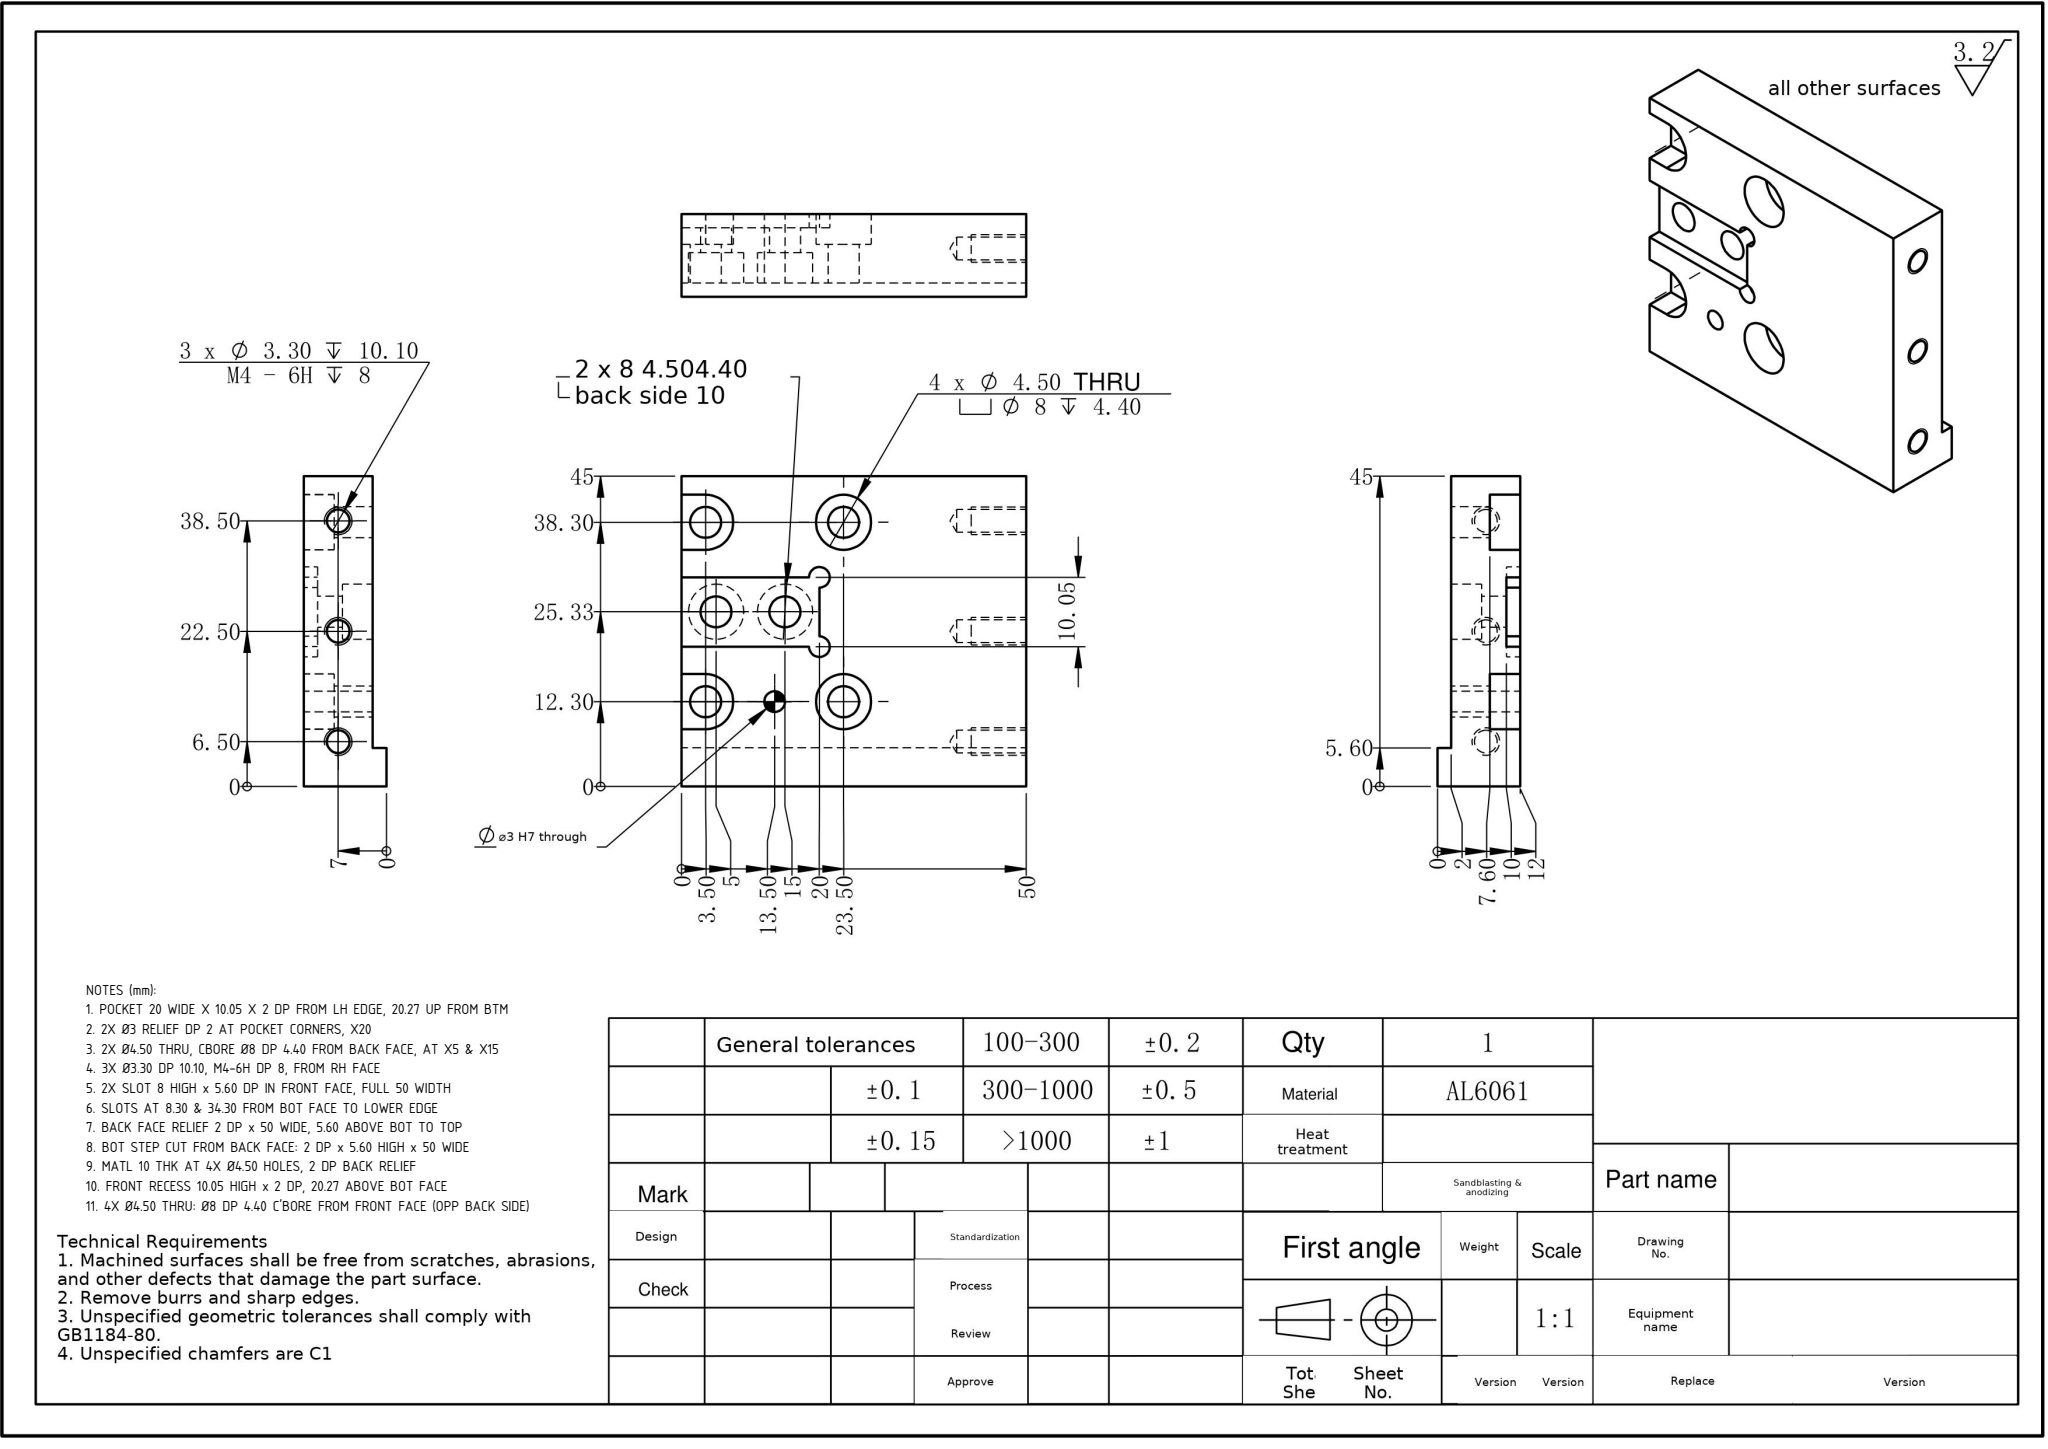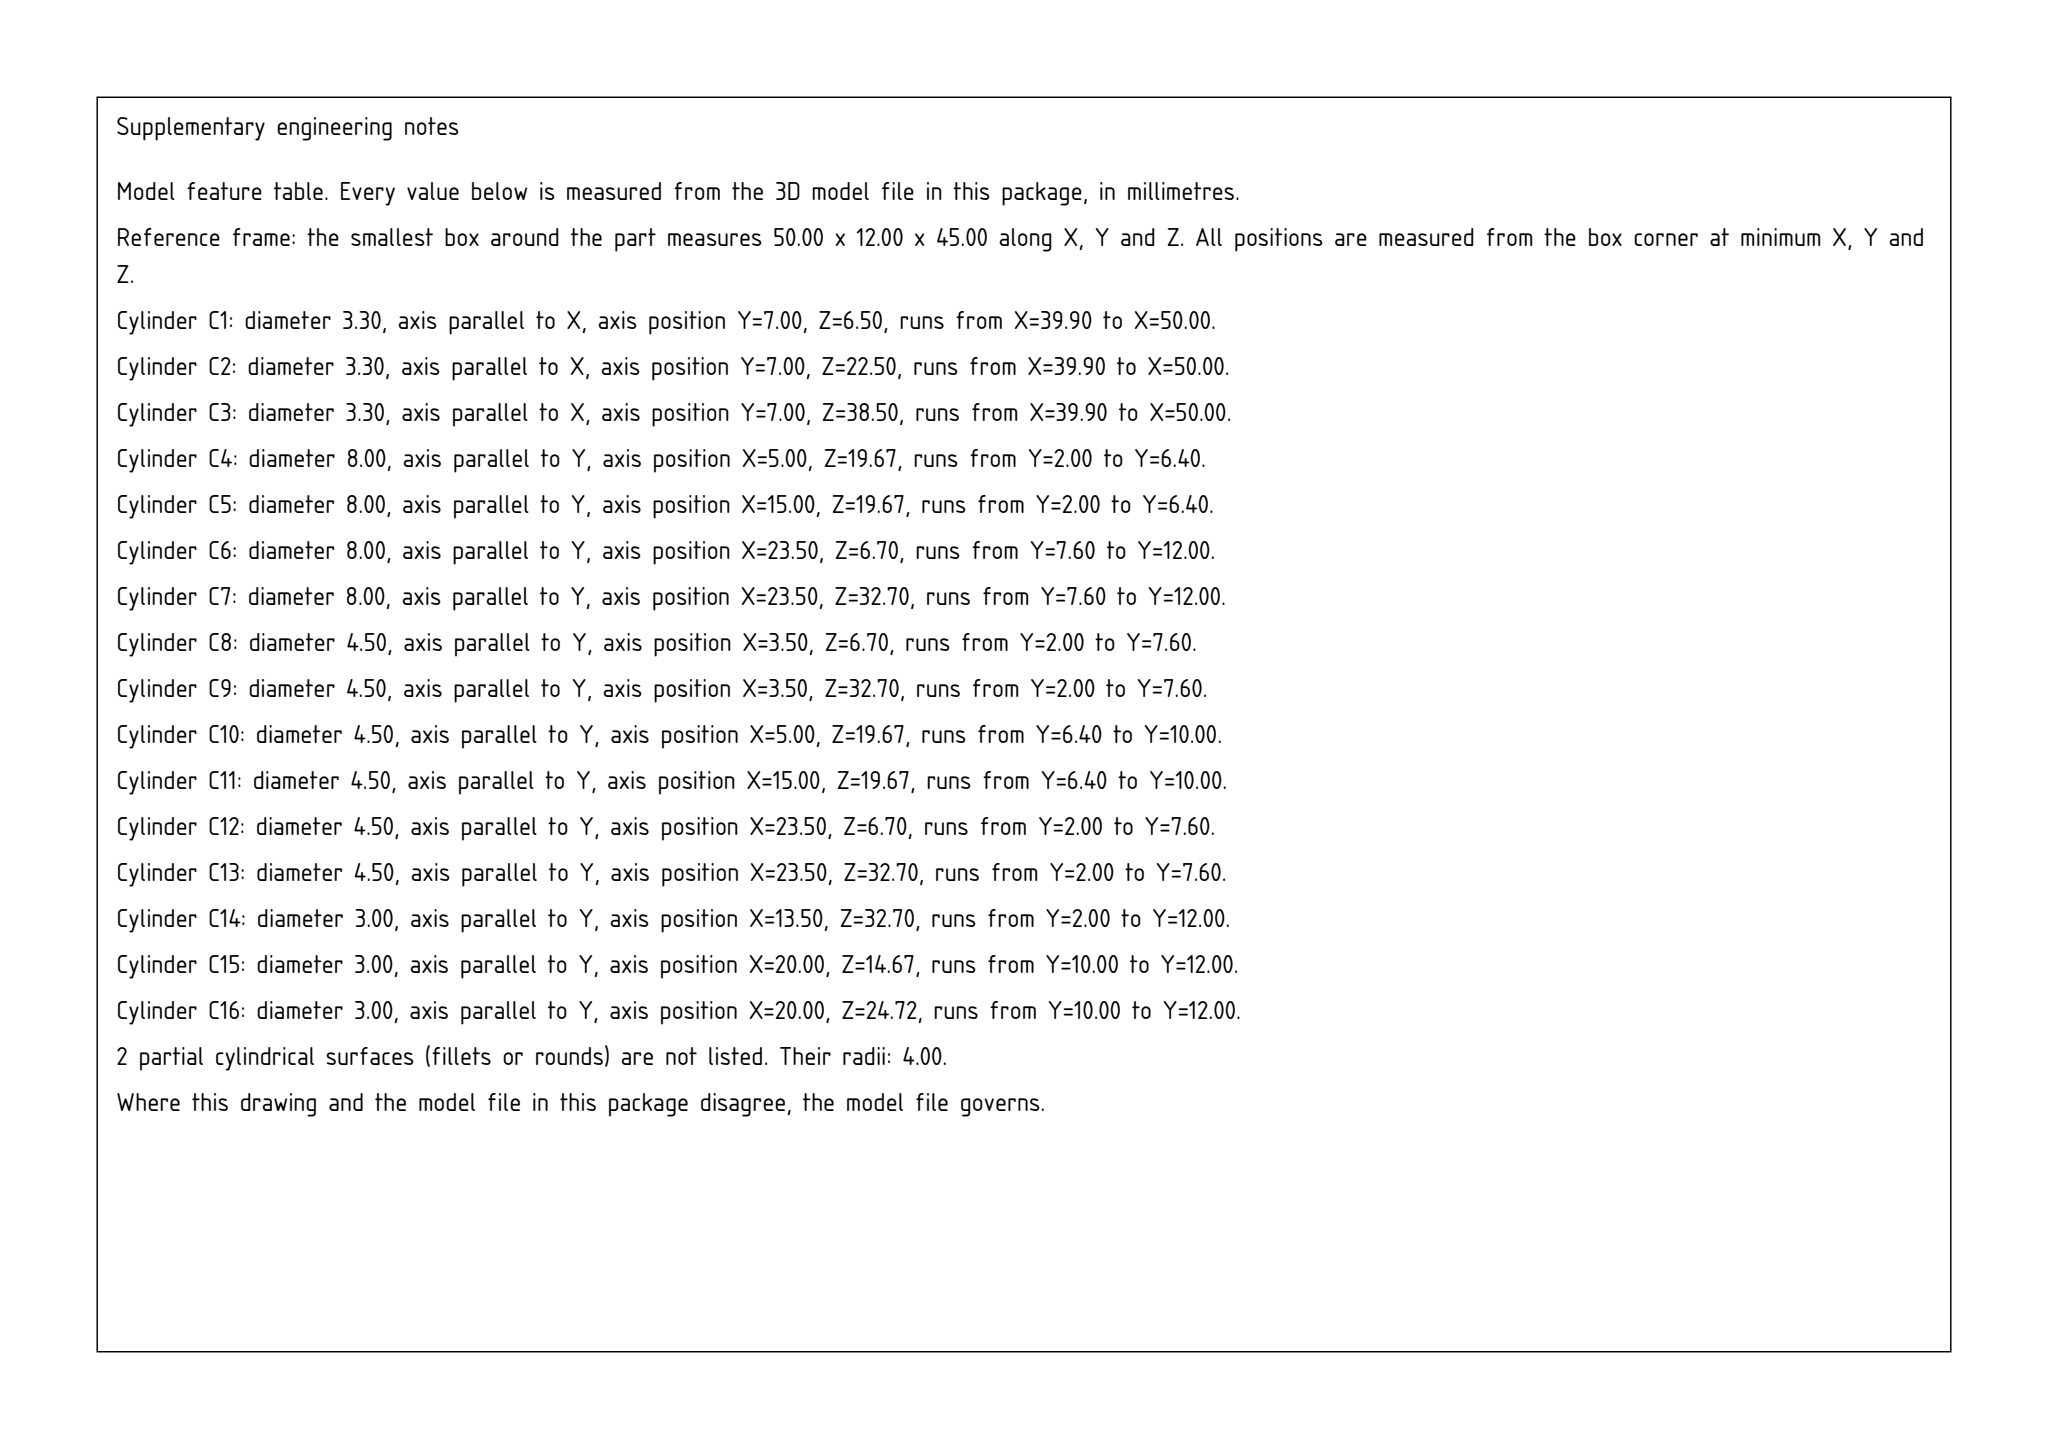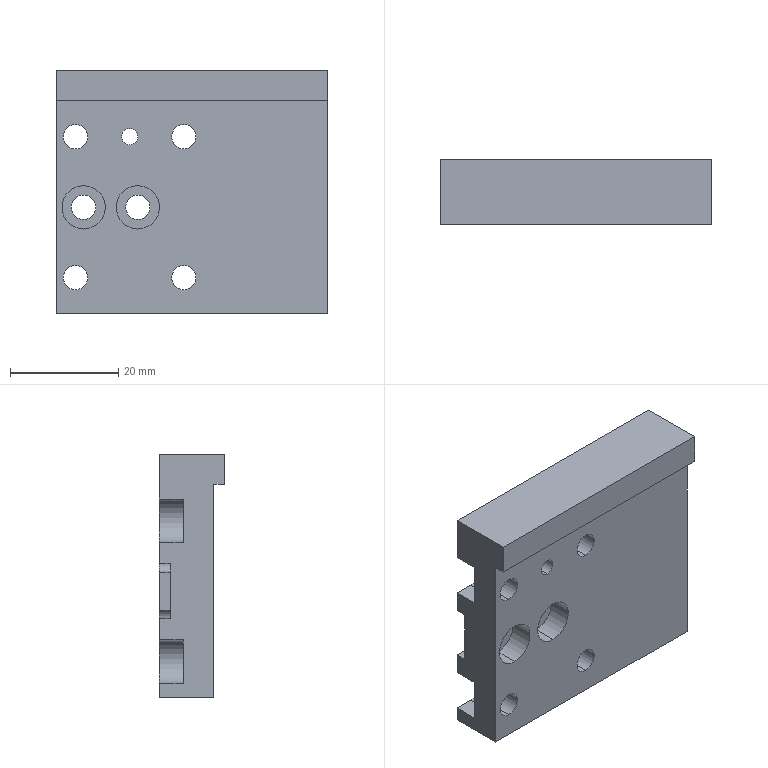Part | SolidWorks | mm | 1 solid | 61 faces | box 50 x 12 x 45 mm | volume 20475 mm3 | cylinder 33 | plane 22 | cone 6 | commonest cylinder face diameters 4.5 x12 8 x10 3.3 x6 3 x5
Drawing notes:
POCKET 20 WIDE X 10.05 X 2 DP FROM LH EDGE, 20.27 UP FROM BTM | from the solid: x planes 0 & 20; z planes 14.68 & 24.73 (10.05 apart, 20.27 up in drawing frame); y planes 10 & 12 = 2 deep
2X Ø3 RELIEF DP 2 AT POCKET CORNERS, X20 | from the solid: cylinders Ø3 axis y at (20,14.68) & (20,24.73), length 2, at pocket end face x=20
2X Ø4.50 THRU, CBORE Ø8 DP 4.40 FROM BACK FACE, AT X5 & X15 | from the solid: Ø4.5 y-axis at (5,19.68) & (15,19.68) len 3.6 (y6.4->10); Ø8 cbore len 4.4 (y2->6.4) from back
3X Ø3.30 DP 10.10, M4-6H DP 8, FROM RH FACE | from the solid: cylinders Ø3.3 axis x at y=7.0, z=6.5/22.5/38.5, length 10.1; cones 118° ref dia 3.3; no slot faces at x>20
2X SLOT 8 HIGH x 5.60 DP IN FRONT FACE, FULL 50 WIDTH | from the solid: z planes 2.7/10.7 and 28.7/36.7 (8 apart); floor plane y=6.4 = 12-6.4 = 5.60 deep from front face y=12; bbox x=50
SLOTS AT 8.30 & 34.30 FROM BOT FACE TO LOWER EDGE | from the solid: drawing height = 45 - model z: z=36.7 -> 8.30, z=10.7 -> 34.30 (slot lower edges), tops at 16.30 & 42.30
BACK FACE RELIEF 2 DP x 50 WIDE, 5.60 ABOVE BOT TO TOP | from the solid: y plane 2.0 vs back face y=0 (2 deep); z plane 39.4 -> 45-39.4 = 5.60 above bottom; x 0 to 50
BOT STEP CUT FROM BACK FACE: 2 DP x 5.60 HIGH x 50 WIDE | from the solid: full 12 thk retained only below z plane 39.4 (=5.60 from bottom); relief floor y=2.0
MATL 10 THK AT 4X Ø4.50 HOLES, 2 DP BACK RELIEF | from the solid: Ø8 c'bore len 4.4 (y=12 to 7.6) + Ø4.5 len 5.6 (y=7.6 to 2.0) = 10 total at x=3.5/23.5, z=6.7/32.7
FRONT RECESS 10.05 HIGH x 2 DP, 20.27 ABOVE BOT FACE | from the solid: z planes 14.68 & 24.73 (10.05 apart) -> 20.27 to 30.32 from bottom; floor y=10 = 2 deep from y=12
4X Ø4.50 THRU: Ø8 DP 4.40 C'BORE FROM FRONT FACE (OPP BACK SIDE) | from the solid: Corner holes x3.5/23.5, z6.7/32.7: Ø4.5 len 5.6 + Ø8 len 4.4 = 10 thk (y2 to y12); cbore floor plane y=7.6 (count 4) => bored from y=12 front face, while 2X holes at x5/x15 have floor y=6.4 (count 2) = back side
build123d program:
from build123d import *

# Parameters (mm, degrees)
SKETCH1_W                                       = 50
SKETCH1_H                                       = 45
BOSS_EXTRUDE1_DEPTH                             = 5
SKETCH2_W                                       = 50
SKETCH2_H                                       = 5.6
BOSS_EXTRUDE2_DEPTH                             = 2
M4_TAPPED_HOLE1_D                               = 3.3
M4_TAPPED_HOLE1_DEPTH                           = 10.1
M4_TAPPED_HOLE1_TIP                             = 0.9914
M4_HEX_SOCKET_HEAD_CAP_SCREW_CBORE1_D           = 4.5
M4_HEX_SOCKET_HEAD_CAP_SCREW_CBORE1_CBORE_D     = 8
M4_HEX_SOCKET_HEAD_CAP_SCREW_CBORE1_CBORE_DEPTH = 4.4
SKETCH7_R                                       = 1.5
CUT_EXTRUDE1_DEPTH                              = 36.711
CUT_EXTRUDE2_DEPTH                              = 4.4
SKETCH9_W                                       = 20
SKETCH9_H                                       = 10.05
CUT_EXTRUDE3_DEPTH                              = 2
SKETCH10_R                                      = 1.5
CUT_EXTRUDE4_DEPTH                              = 2
M4_HEX_SOCKET_HEAD_CAP_SCREW_CBORE3_D           = 4.5
M4_HEX_SOCKET_HEAD_CAP_SCREW_CBORE3_DEPTH       = 10
M4_HEX_SOCKET_HEAD_CAP_SCREW_CBORE3_CBORE_D     = 8
M4_HEX_SOCKET_HEAD_CAP_SCREW_CBORE3_CBORE_DEPTH = 4.4
M4_HEX_SOCKET_HEAD_CAP_SCREW_CBORE3_TIP         = 1.352


with BuildPart() as part:
    # Sketch1 → Boss-Extrude1 (new, symmetric)
    with BuildSketch(Plane(origin=(0, 0, 0), x_dir=(1, 0, 0), z_dir=(0, 1, 0))):
        Rectangle(SKETCH1_W, SKETCH1_H)
    extrude(amount=BOSS_EXTRUDE1_DEPTH, both=True)

    # Sketch2 → Boss-Extrude2 (add)
    with BuildSketch(Plane.XZ.offset(5)):
        with Locations((0, 19.7)):
            Rectangle(SKETCH2_W, SKETCH2_H)
    extrude(amount=BOSS_EXTRUDE2_DEPTH)

    # M4 Tapped Hole1
    with Locations(Plane(origin=(25, 0, 0), x_dir=(0, 0, -1), z_dir=(1, 0, 0))):
        with Locations((16, 0), (0, 0), (-16, 0)):
            Hole(M4_TAPPED_HOLE1_D / 2, depth=M4_TAPPED_HOLE1_DEPTH)
            with Locations((0, 0, -(M4_TAPPED_HOLE1_DEPTH + M4_TAPPED_HOLE1_TIP / 2))):  # 118° drill point
                Cone(0, M4_TAPPED_HOLE1_D / 2, M4_TAPPED_HOLE1_TIP, mode=Mode.SUBTRACT)

    # M4 Hex Socket Head Cap Screw CBORE1 (through all)
    with Locations(Plane(origin=(0, 5, 0), x_dir=(1, 0, 0), z_dir=(0, 1, 0))):
        with Locations((-21.5, 15.8), (-1.5, 15.8), (-21.5, -10.2), (-1.5, -10.2)):
            CounterBoreHole(M4_HEX_SOCKET_HEAD_CAP_SCREW_CBORE1_D / 2, M4_HEX_SOCKET_HEAD_CAP_SCREW_CBORE1_CBORE_D / 2, M4_HEX_SOCKET_HEAD_CAP_SCREW_CBORE1_CBORE_DEPTH)

    # Sketch7 → Cut-Extrude1 (cut, through all)
    with BuildSketch(Plane(origin=(0, 5, 0), x_dir=(1, 0, 0), z_dir=(0, 1, 0))):
        with Locations(Location((-11.5, -10.2, 0), (0, 0, 270))):
            Circle(SKETCH7_R)
    extrude(amount=-CUT_EXTRUDE1_DEPTH, mode=Mode.SUBTRACT)

    # Sketch8 → Cut-Extrude2 (cut)
    with BuildSketch(Plane(origin=(0, 5, 0), x_dir=(1, 0, 0), z_dir=(0, 1, 0))):
        with BuildLine():
            Line((-21.5, 11.8), (-31.5, 11.8))
            ThreePointArc((-31.5, 11.8), (-35.5, 15.8), (-31.5, 19.8))
            Line((-31.5, 19.8), (-21.5, 19.8))
            ThreePointArc((-21.5, 19.8), (-17.5, 15.8), (-21.5, 11.8))
        make_face()
        with BuildLine():
            Line((-21.5, -14.2), (-31.5, -14.2))
            ThreePointArc((-31.5, -14.2), (-35.5, -10.2), (-31.5, -6.2))
            Line((-31.5, -6.2), (-21.5, -6.2))
            ThreePointArc((-21.5, -6.2), (-17.5, -10.2), (-21.5, -14.2))
        make_face()
    extrude(amount=-CUT_EXTRUDE2_DEPTH, mode=Mode.SUBTRACT)

    # Sketch9 → Cut-Extrude3 (cut)
    with BuildSketch(Plane(origin=(0, 5, 0), x_dir=(1, 0, 0), z_dir=(0, 1, 0))):
        with Locations((-15, 2.8)):
            Rectangle(SKETCH9_W, SKETCH9_H)
    extrude(amount=-CUT_EXTRUDE3_DEPTH, mode=Mode.SUBTRACT)

    # Sketch10 → Cut-Extrude4 (cut)
    with BuildSketch(Plane(origin=(0, 5, 0), x_dir=(1, 0, 0), z_dir=(0, 1, 0))):
        with Locations((-5, 7.825)):
            Circle(SKETCH10_R)
        with Locations((-5, -2.225)):
            Circle(SKETCH10_R)
    extrude(amount=-CUT_EXTRUDE4_DEPTH, mode=Mode.SUBTRACT)

    # M4 Hex Socket Head Cap Screw CBORE3
    with Locations(Plane(origin=(0, -5, 0), x_dir=(-1, 0, 0), z_dir=(0, -1, 0))):
        with Locations((20, 2.825), (10, 2.825)):
            CounterBoreHole(M4_HEX_SOCKET_HEAD_CAP_SCREW_CBORE3_D / 2, M4_HEX_SOCKET_HEAD_CAP_SCREW_CBORE3_CBORE_D / 2, M4_HEX_SOCKET_HEAD_CAP_SCREW_CBORE3_CBORE_DEPTH, depth=M4_HEX_SOCKET_HEAD_CAP_SCREW_CBORE3_DEPTH)
            with Locations((0, 0, -(M4_HEX_SOCKET_HEAD_CAP_SCREW_CBORE3_DEPTH + M4_HEX_SOCKET_HEAD_CAP_SCREW_CBORE3_TIP / 2))):  # 118° drill point
                Cone(0, M4_HEX_SOCKET_HEAD_CAP_SCREW_CBORE3_D / 2, M4_HEX_SOCKET_HEAD_CAP_SCREW_CBORE3_TIP, mode=Mode.SUBTRACT)


solid = part.part